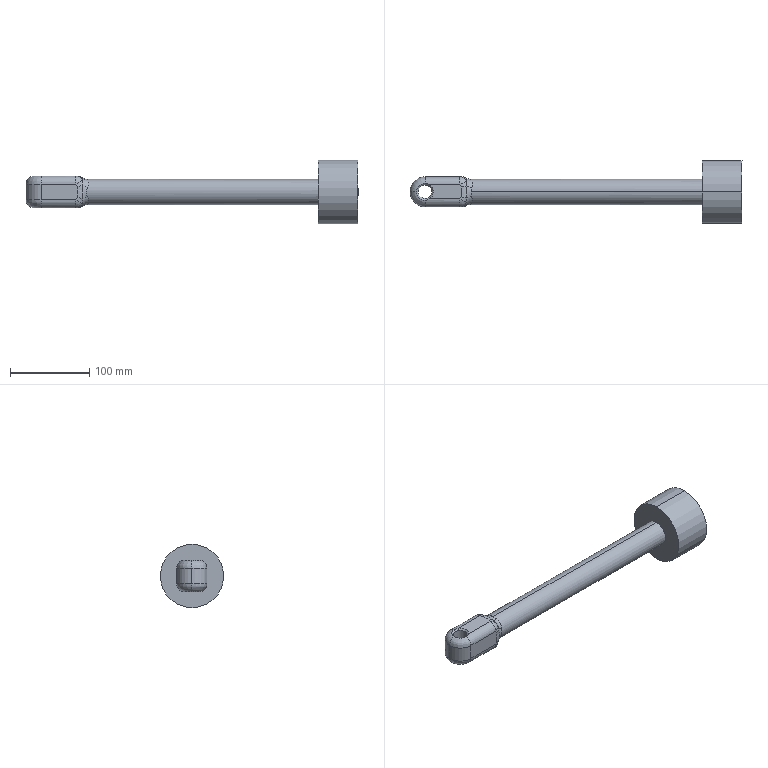Component | SolidWorks | CylinderPistonRod-2 | 1 solid | 56 faces | volume 576423 mm3 | spline 24 | cylinder 12 | cone 6 | plane 6 | torus 4 | sphere 4 | commonest cylinder face diameters 20 x4 17 x2 38 x2 32 x2 80 x2 | material 45